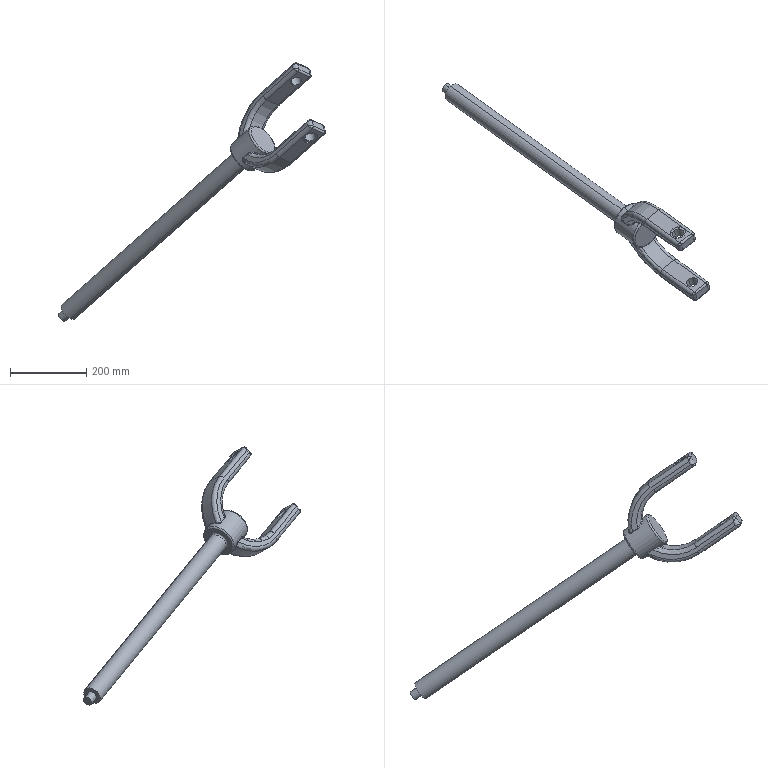Component | SolidWorks | Strut-1 | 1 solid | 90 faces | volume 2736853 mm3 | cylinder 38 | spline 20 | plane 18 | torus 14 | commonest cylinder face diameters 20 x12 40 x4 30 x4 10 x4 5 x4 50 x2 25 x2 90 x2 | material 201.0-T7 Insulated Mold Casting (SS)